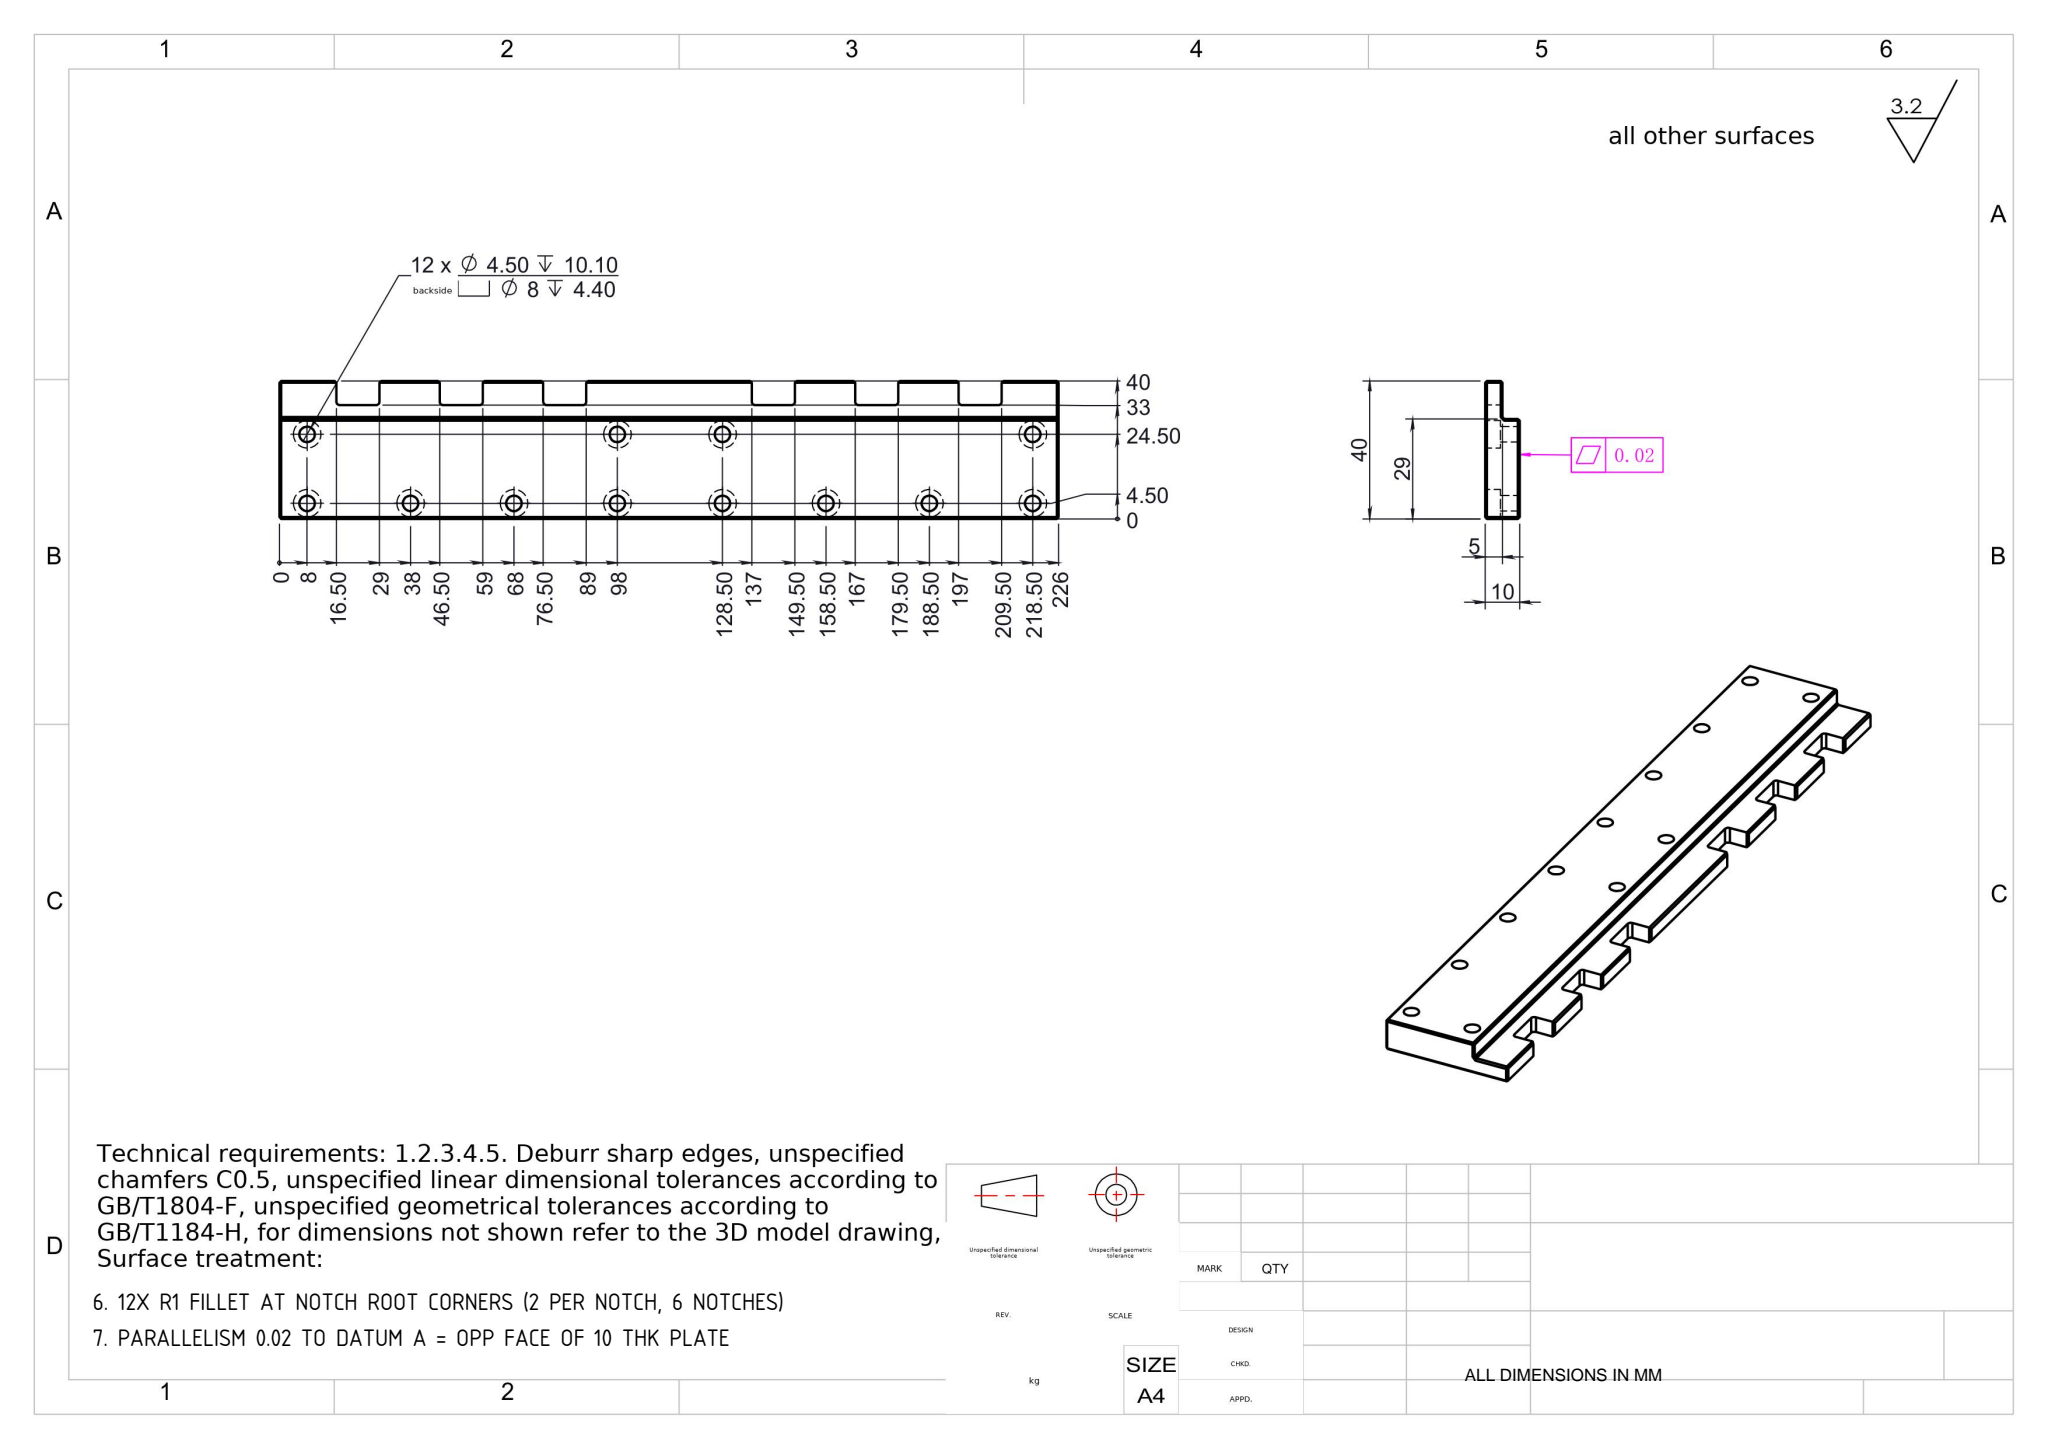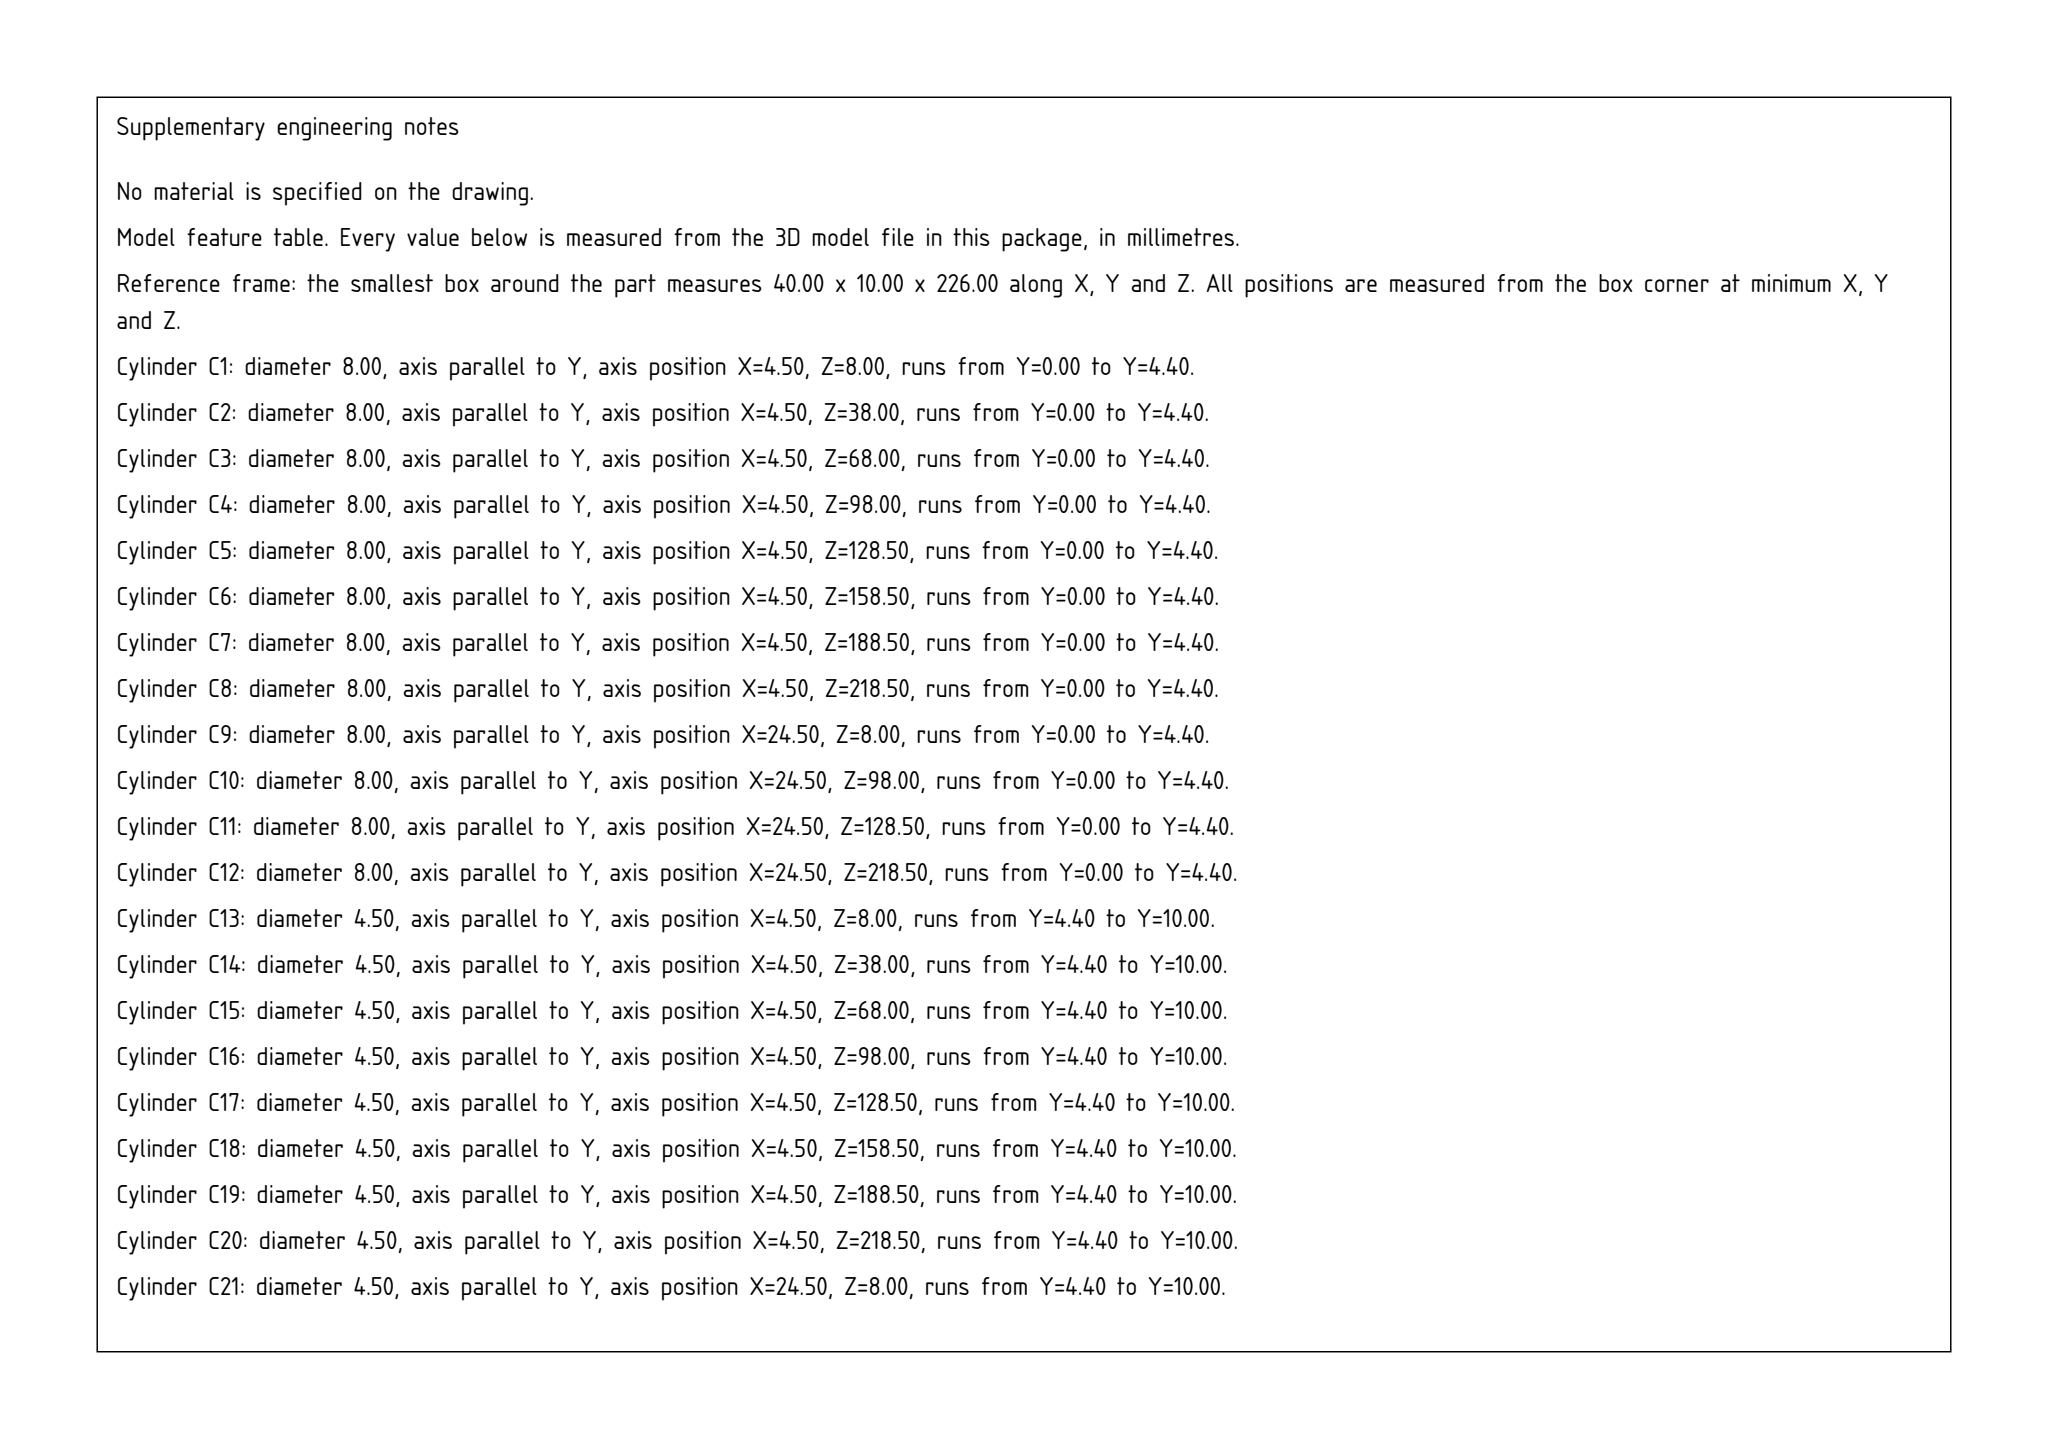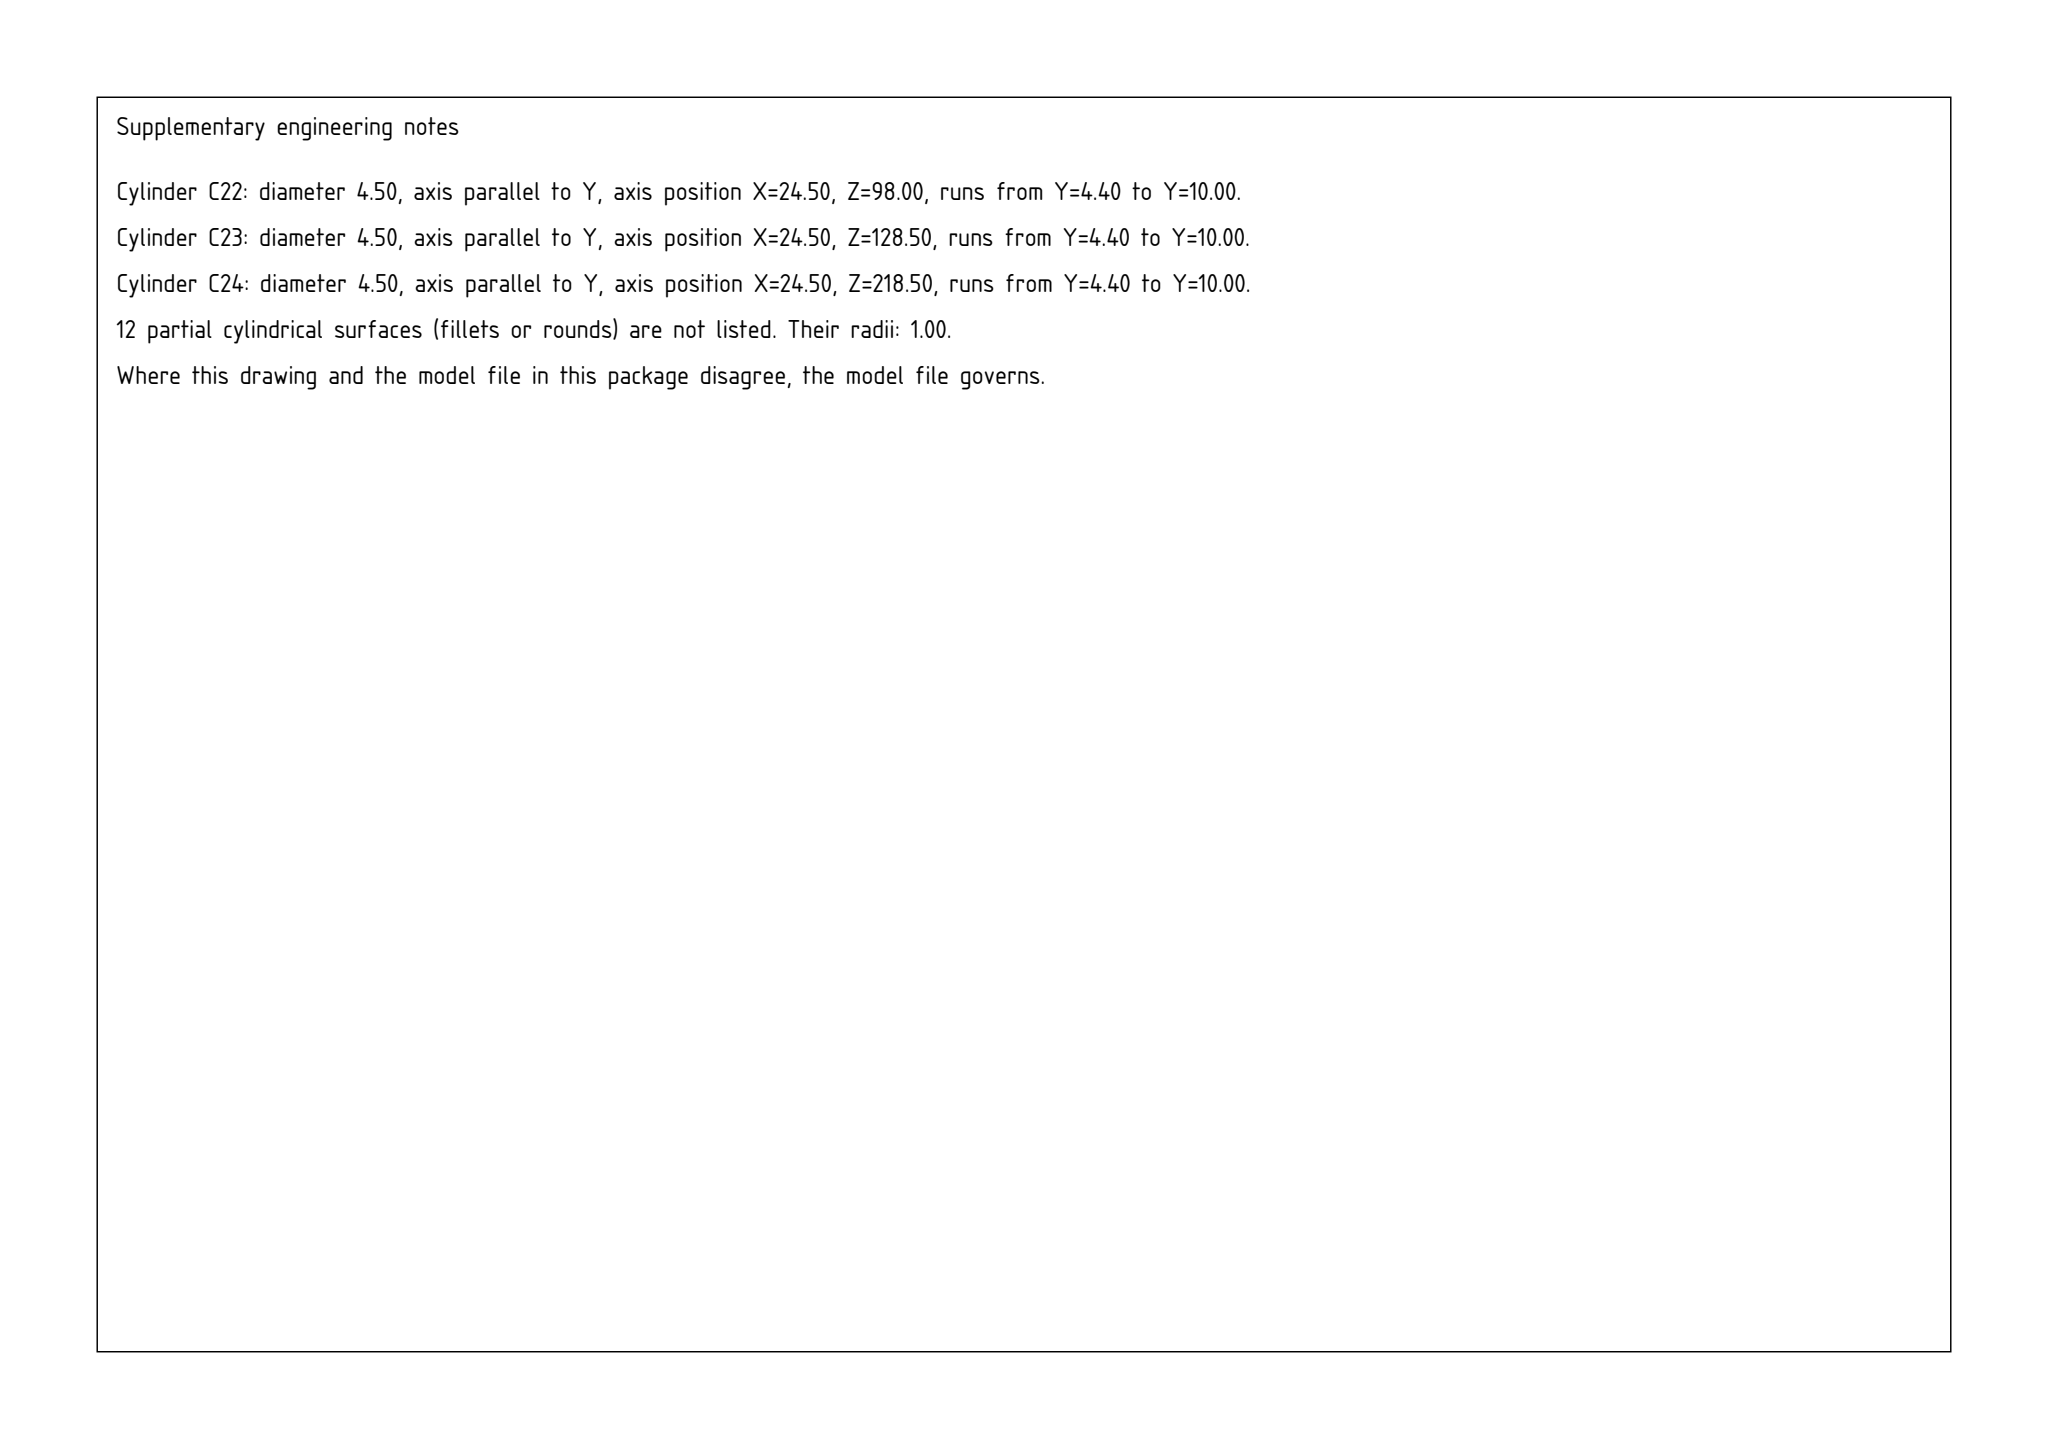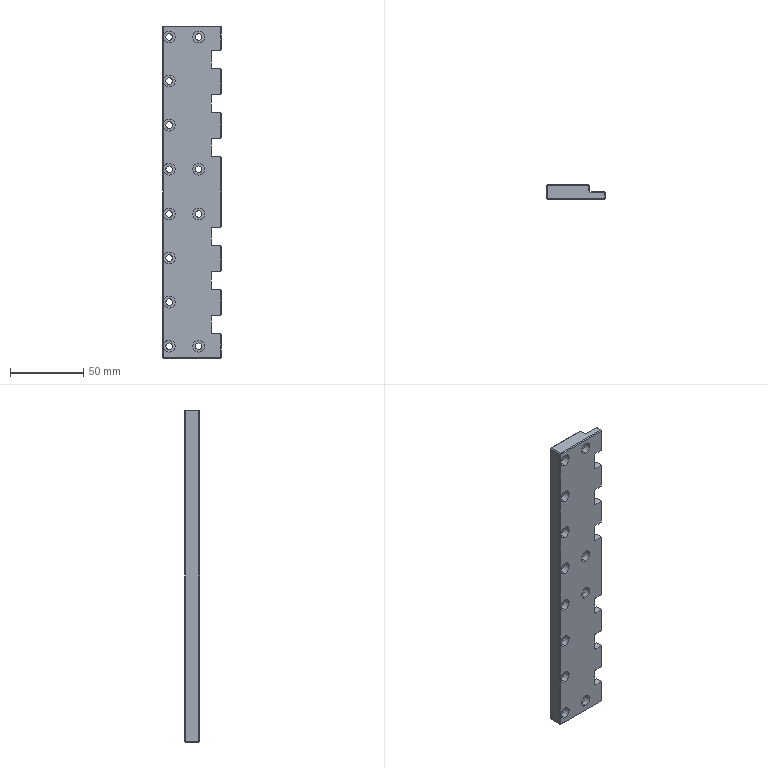Part | SolidWorks | mm | material Black POM | 1 solid | 158 faces | box 40 x 10 x 226 mm | volume 71510 mm3 | plane 98 | cylinder 60 | commonest cylinder face diameters 8 x24 4.5 x24 2 x12
Drawing notes:
12X R1 FILLET AT NOTCH ROOT CORNERS (2 PER NOTCH, 6 NOTCHES) | from the solid: 12 concave arcs dia 2.0, axis y, at x=34 (1 mm off notch floor x=33), z=17.5/28/47.5/58/77.5/88/138/148.5/168/178.5/198/208.5, 90 deg, y 0-5
PARALLELISM 0.02 TO DATUM A = OPP FACE OF 10 THK PLATE | from the solid: Planes y=0 (area 7687, x0.5-39.5 x z0.5-225.5) and y=10 (area 6109, x0.5-28.5) are the two parallel outer faces of the 10 thk body; toleranced face in side view is the y=10 face, datum is the full y=0 mounting face
build123d program:
from build123d import *

# Parameters (mm, degrees)
SKETCH2_W                                       = 40
SKETCH2_H                                       = 226
BOSS_EXTRUDE1_DEPTH                             = 5
SKETCH3_W                                       = 11
SKETCH3_H                                       = 5
CUT_EXTRUDE1_DEPTH                              = 227.938
CHAMFER1_SIZE                                   = 0.5
SKETCH5_W                                       = 7
SKETCH5_H                                       = 12.5
CUT_EXTRUDE3_DEPTH                              = 20
FILLET1_R                                       = 1
CHAMFER2_SIZE                                   = 0.5
LPATTERN2_COUNT                                 = 2
LPATTERN2_PITCH                                 = 120.5
FILLET1_OF_LPATTERN2_R                          = 1
CHAMFER2_OF_LPATTERN2_SIZE                      = 0.5
M4_HEX_SOCKET_HEAD_CAP_SCREW_CBORE1_D           = 4.5
M4_HEX_SOCKET_HEAD_CAP_SCREW_CBORE1_DEPTH       = 10.1
M4_HEX_SOCKET_HEAD_CAP_SCREW_CBORE1_CBORE_D     = 8
M4_HEX_SOCKET_HEAD_CAP_SCREW_CBORE1_CBORE_DEPTH = 4.4
M4_HEX_SOCKET_HEAD_CAP_SCREW_CBORE1_TIP         = 1.352


with BuildPart() as part:
    # Sketch2 → Boss-Extrude1 (new, symmetric)
    with BuildSketch(Plane(origin=(0, 0, 0), x_dir=(1, 0, 0), z_dir=(0, 1, 0))):
        Rectangle(SKETCH2_W, SKETCH2_H)
    extrude(amount=BOSS_EXTRUDE1_DEPTH, both=True)

    # Sketch3 → Cut-Extrude1 (cut, through all)
    with BuildSketch(Plane.XY.offset(113)):
        with Locations((14.5, 2.5)):
            Rectangle(SKETCH3_W, SKETCH3_H)
    extrude(amount=-CUT_EXTRUDE1_DEPTH, mode=Mode.SUBTRACT)

    # Chamfer1
    chamfer1_edges = [part.edges().sort_by_distance(p)[0] for p in [
        (-20, 5, 0),
        (-5.5, 5, -113),
        (20, -2.5, 113),
        (20, -2.5, -113),
        (-5.5, 5, 113),
        (14.5, 0, -113),
        (20, 0, 0),
        (9, 2.5, -113),
        (9, 0, 0),
        (9, 5, 0),
        (9, 2.5, 113),
        (14.5, 0, 113),
        (0, -5, 113),
        (-20, -5, 0),
        (0, -5, -113),
        (20, -5, 0),
        (-20, 0, 113),
        (-20, 0, -113),
    ]]
    chamfer(chamfer1_edges, length=CHAMFER1_SIZE)

    # Sketch5 → Cut-Extrude3 (cut)
    with BuildSketch(Plane(origin=(0, 0, 0), x_dir=(1, 0, 0), z_dir=(0, 1, 0))):
        with Locations((16.5, 30.25)):
            Rectangle(SKETCH5_W, SKETCH5_H)
        with Locations((16.5, 60.25)):
            Rectangle(SKETCH5_W, SKETCH5_H)
        with Locations((16.5, 90.25)):
            Rectangle(SKETCH5_W, SKETCH5_H)
    cut_extrude3 = extrude(amount=-CUT_EXTRUDE3_DEPTH, mode=Mode.SUBTRACT)

    # Fillet1
    fillet1_edges = [part.edges().sort_by_distance(p)[0] for p in [
        (13, -2.5, -24),
        (13, -2.5, -36.5),
        (13, -2.5, -54),
        (13, -2.5, -66.5),
        (13, -2.5, -84),
        (13, -2.5, -96.5),
    ]]
    fillet(fillet1_edges, radius=FILLET1_R)

    # Chamfer2
    chamfer2_edges = [part.edges().sort_by_distance(p)[0] for p in [
        (20, -2.5, -96.5),
        (20, -2.5, -84),
        (20, -2.5, -66.5),
        (20, -2.5, -54),
        (20, -2.5, -36.5),
        (20, -2.5, -24),
    ]]
    chamfer(chamfer2_edges, length=CHAMFER2_SIZE)

    # LPattern2: Cut-Extrude3 ×2
    with Locations(*[(0, 0, i * LPATTERN2_PITCH) for i in range(1, LPATTERN2_COUNT)]):
        add(cut_extrude3, mode=Mode.SUBTRACT)

    # Fillet1 of LPattern2
    fillet1_of_lpattern2_edges = [part.edges().sort_by_distance(p)[0] for p in [
        (13, -2.5, 96.5),
        (13, -2.5, 84),
        (13, -2.5, 66.5),
        (13, -2.5, 54),
        (13, -2.5, 36.5),
        (13, -2.5, 24),
    ]]
    fillet(fillet1_of_lpattern2_edges, radius=FILLET1_OF_LPATTERN2_R)

    # Chamfer2 of LPattern2
    chamfer2_of_lpattern2_edges = [part.edges().sort_by_distance(p)[0] for p in [
        (20, -2.5, 24),
        (20, -2.5, 36.5),
        (20, -2.5, 54),
        (20, -2.5, 66.5),
        (20, -2.5, 84),
        (20, -2.5, 96.5),
    ]]
    chamfer(chamfer2_of_lpattern2_edges, length=CHAMFER2_OF_LPATTERN2_SIZE)

    # M4 Hex Socket Head Cap Screw CBORE1
    with Locations(Plane(origin=(0, -5, 0), x_dir=(-1, 0, 0), z_dir=(0, -1, 0))):
        with Locations((15.5, 105), (-4.5, 105), (15.5, 75), (15.5, 45), (15.5, 15), (-4.5, 15), (15.5, -15.5), (-4.5, -15.5), (15.5, -45.5), (15.5, -75.5), (15.5, -105.5), (-4.5, -105.5)):
            CounterBoreHole(M4_HEX_SOCKET_HEAD_CAP_SCREW_CBORE1_D / 2, M4_HEX_SOCKET_HEAD_CAP_SCREW_CBORE1_CBORE_D / 2, M4_HEX_SOCKET_HEAD_CAP_SCREW_CBORE1_CBORE_DEPTH, depth=M4_HEX_SOCKET_HEAD_CAP_SCREW_CBORE1_DEPTH)
            with Locations((0, 0, -(M4_HEX_SOCKET_HEAD_CAP_SCREW_CBORE1_DEPTH + M4_HEX_SOCKET_HEAD_CAP_SCREW_CBORE1_TIP / 2))):  # 118° drill point
                Cone(0, M4_HEX_SOCKET_HEAD_CAP_SCREW_CBORE1_D / 2, M4_HEX_SOCKET_HEAD_CAP_SCREW_CBORE1_TIP, mode=Mode.SUBTRACT)


solid = part.part